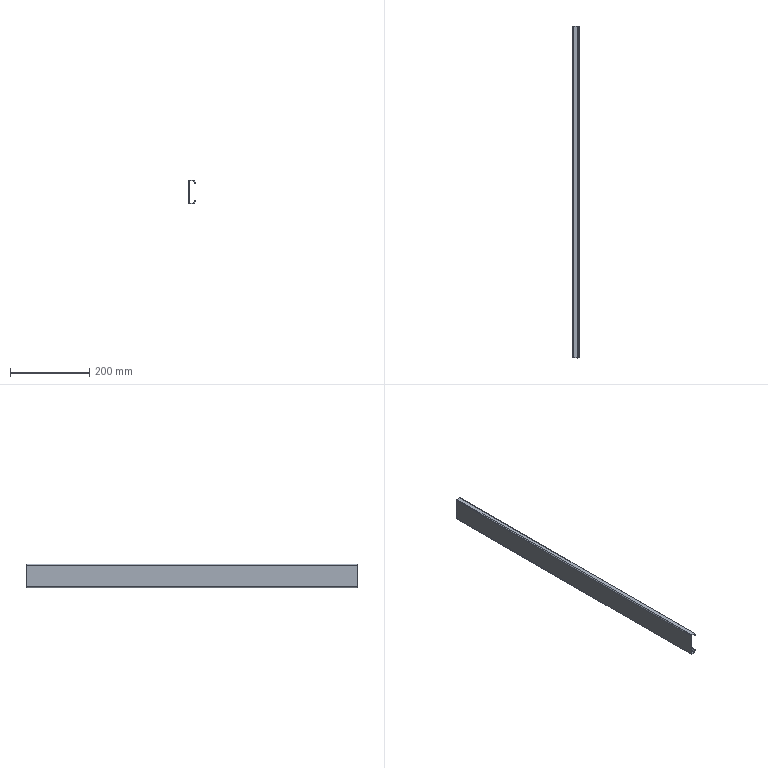Component | SolidWorks | MiddleCrossbar400AType40001100-3 | 1 solid | 54 faces | volume 134842 mm3 | plane 42 | cylinder 12 | commonest cylinder face diameters 4.473 x4 1.473 x4 3.1 x2 0.1 x2